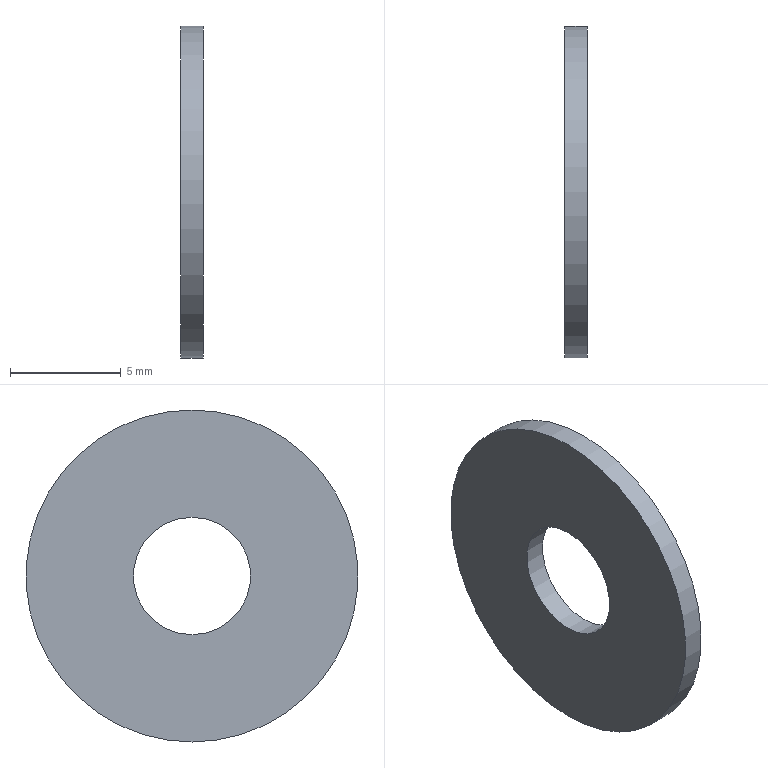Component | NX | GB-T96_1-2002_M5 | 1 solid | 4 faces | box 1 x 15 x 15 mm | volume 155 mm3 | cylinder 2 | plane 2 | commonest cylinder face diameters 15 x1 5.3 x1
STEP:
#1=CARTESIAN_POINT('',(0.,0.,0.));
#2=DIRECTION('',(0.,0.,1.));
#3=DIRECTION('',(1.,0.,0.));
#4=AXIS2_PLACEMENT_3D('',#1,#2,#3);
#5=CARTESIAN_POINT('',(16.,-0.,39.5));
#6=VERTEX_POINT('',#5);
#7=CARTESIAN_POINT('',(16.,-0.,32.));
#8=DIRECTION('',(-1.,0.,0.));
#9=DIRECTION('',(0.,0.,1.));
#10=AXIS2_PLACEMENT_3D('',#7,#8,#9);
#11=CIRCLE('',#10,7.5);
#12=CARTESIAN_POINT('',(16.,-0.,32.));
#13=DIRECTION('',(1.,0.,0.));
#14=DIRECTION('',(0.,0.,-1.));
#15=AXIS2_PLACEMENT_3D('',#12,#13,#14);
#16=CYLINDRICAL_SURFACE('',#15,7.5);
#17=CARTESIAN_POINT('',(9.425,0.));
#18=DIRECTION('',(-1.,0.));
#19=VECTOR('',#18,1.);
#20=LINE('',#17,#19);
#21=(GEOMETRIC_REPRESENTATION_CONTEXT(2)PARAMETRIC_REPRESENTATION_CONTEXT()REPRESENTATION_CONTEXT('',''));
#22=DEFINITIONAL_REPRESENTATION('',(#20),#21);
#23=PCURVE('',#16,#22);
#24=CARTESIAN_POINT('',(16.,-0.,32.));
#25=DIRECTION('',(-1.,0.,0.));
#26=DIRECTION('',(0.,0.,1.));
#27=AXIS2_PLACEMENT_3D('',#24,#25,#26);
#28=PLANE('',#27);
#29=CARTESIAN_POINT('',(0.,0.));
#30=DIRECTION('',(1.,0.));
#31=AXIS2_PLACEMENT_2D('',#29,#30);
#32=CIRCLE('',#31,7.5);
#33=(GEOMETRIC_REPRESENTATION_CONTEXT(2)PARAMETRIC_REPRESENTATION_CONTEXT()REPRESENTATION_CONTEXT('',''));
#34=DEFINITIONAL_REPRESENTATION('',(#32),#33);
#35=PCURVE('',#28,#34);
#36=SURFACE_CURVE('',#11,(#23,#35),.PCURVE_S1.);
#37=EDGE_CURVE('',#6,#6,#36,.T.);
#38=ORIENTED_EDGE('',*,*,#37,.F.);
#39=CARTESIAN_POINT('',(17.,-0.,39.5));
#40=VERTEX_POINT('',#39);
#41=CARTESIAN_POINT('',(16.,-0.,39.5));
#42=CARTESIAN_POINT('',(17.,-0.,39.5));
#43=B_SPLINE_CURVE_WITH_KNOTS('',1,(#41,#42),.UNSPECIFIED.,.F.,.F.,(2,2),(0.,1.),.PIECEWISE_BEZIER_KNOTS.);
#44=CARTESIAN_POINT('',(9.425,0.));
#45=DIRECTION('',(0.,1.));
#46=VECTOR('',#45,1.);
#47=LINE('',#44,#46);
#48=(GEOMETRIC_REPRESENTATION_CONTEXT(2)PARAMETRIC_REPRESENTATION_CONTEXT()REPRESENTATION_CONTEXT('',''));
#49=DEFINITIONAL_REPRESENTATION('',(#47),#48);
#50=PCURVE('',#16,#49);
#51=CARTESIAN_POINT('',(3.142,0.));
#52=DIRECTION('',(0.,1.));
#53=VECTOR('',#52,1.);
#54=LINE('',#51,#53);
#55=(GEOMETRIC_REPRESENTATION_CONTEXT(2)PARAMETRIC_REPRESENTATION_CONTEXT()REPRESENTATION_CONTEXT('',''));
#56=DEFINITIONAL_REPRESENTATION('',(#54),#55);
#57=PCURVE('',#16,#56);
#58=SEAM_CURVE('',#43,(#50,#57),.PCURVE_S1.);
#59=EDGE_CURVE('',#6,#40,#58,.T.);
#60=ORIENTED_EDGE('',*,*,#59,.T.);
#61=CARTESIAN_POINT('',(17.,-0.,32.));
#62=DIRECTION('',(-1.,0.,0.));
#63=DIRECTION('',(0.,0.,1.));
#64=AXIS2_PLACEMENT_3D('',#61,#62,#63);
#65=CIRCLE('',#64,7.5);
#66=CARTESIAN_POINT('',(9.425,1.));
#67=DIRECTION('',(-1.,0.));
#68=VECTOR('',#67,1.);
#69=LINE('',#66,#68);
#70=(GEOMETRIC_REPRESENTATION_CONTEXT(2)PARAMETRIC_REPRESENTATION_CONTEXT()REPRESENTATION_CONTEXT('',''));
#71=DEFINITIONAL_REPRESENTATION('',(#69),#70);
#72=PCURVE('',#16,#71);
#73=CARTESIAN_POINT('',(17.,-0.,32.));
#74=DIRECTION('',(-1.,0.,0.));
#75=DIRECTION('',(0.,0.,1.));
#76=AXIS2_PLACEMENT_3D('',#73,#74,#75);
#77=PLANE('',#76);
#78=CARTESIAN_POINT('',(0.,0.));
#79=DIRECTION('',(1.,0.));
#80=AXIS2_PLACEMENT_2D('',#78,#79);
#81=CIRCLE('',#80,7.5);
#82=(GEOMETRIC_REPRESENTATION_CONTEXT(2)PARAMETRIC_REPRESENTATION_CONTEXT()REPRESENTATION_CONTEXT('',''));
#83=DEFINITIONAL_REPRESENTATION('',(#81),#82);
#84=PCURVE('',#77,#83);
#85=SURFACE_CURVE('',#65,(#72,#84),.PCURVE_S1.);
#86=EDGE_CURVE('',#40,#40,#85,.T.);
#87=ORIENTED_EDGE('',*,*,#86,.T.);
#88=ORIENTED_EDGE('',*,*,#59,.F.);
#89=EDGE_LOOP('',(#38,#60,#87,#88));
#90=FACE_BOUND('',#89,.T.);
#91=ADVANCED_FACE('',(#90),#16,.T.);
#92=CARTESIAN_POINT('',(16.,-0.,34.65));
#93=VERTEX_POINT('',#92);
#94=CARTESIAN_POINT('',(16.,-0.,32.));
#95=DIRECTION('',(-1.,0.,0.));
#96=DIRECTION('',(0.,0.,1.));
#97=AXIS2_PLACEMENT_3D('',#94,#95,#96);
#98=CIRCLE('',#97,2.65);
#99=CARTESIAN_POINT('',(16.,-0.,32.));
#100=DIRECTION('',(1.,0.,0.));
#101=DIRECTION('',(0.,0.,-1.));
#102=AXIS2_PLACEMENT_3D('',#99,#100,#101);
#103=CYLINDRICAL_SURFACE('',#102,2.65);
#104=CARTESIAN_POINT('',(9.425,0.));
#105=DIRECTION('',(-1.,0.));
#106=VECTOR('',#105,1.);
#107=LINE('',#104,#106);
#108=(GEOMETRIC_REPRESENTATION_CONTEXT(2)PARAMETRIC_REPRESENTATION_CONTEXT()REPRESENTATION_CONTEXT('',''));
#109=DEFINITIONAL_REPRESENTATION('',(#107),#108);
#110=PCURVE('',#103,#109);
#111=CARTESIAN_POINT('',(0.,0.));
#112=DIRECTION('',(1.,0.));
#113=AXIS2_PLACEMENT_2D('',#111,#112);
#114=CIRCLE('',#113,2.65);
#115=(GEOMETRIC_REPRESENTATION_CONTEXT(2)PARAMETRIC_REPRESENTATION_CONTEXT()REPRESENTATION_CONTEXT('',''));
#116=DEFINITIONAL_REPRESENTATION('',(#114),#115);
#117=PCURVE('',#28,#116);
#118=SURFACE_CURVE('',#98,(#110,#117),.PCURVE_S1.);
#119=EDGE_CURVE('',#93,#93,#118,.T.);
#120=ORIENTED_EDGE('',*,*,#119,.F.);
#121=CARTESIAN_POINT('',(17.,-0.,34.65));
#122=VERTEX_POINT('',#121);
#123=CARTESIAN_POINT('',(16.,-0.,34.65));
#124=CARTESIAN_POINT('',(17.,-0.,34.65));
#125=B_SPLINE_CURVE_WITH_KNOTS('',1,(#123,#124),.UNSPECIFIED.,.F.,.F.,(2,2),(0.,1.),.PIECEWISE_BEZIER_KNOTS.);
#126=CARTESIAN_POINT('',(9.425,0.));
#127=DIRECTION('',(0.,1.));
#128=VECTOR('',#127,1.);
#129=LINE('',#126,#128);
#130=(GEOMETRIC_REPRESENTATION_CONTEXT(2)PARAMETRIC_REPRESENTATION_CONTEXT()REPRESENTATION_CONTEXT('',''));
#131=DEFINITIONAL_REPRESENTATION('',(#129),#130);
#132=PCURVE('',#103,#131);
#133=CARTESIAN_POINT('',(3.142,0.));
#134=DIRECTION('',(0.,1.));
#135=VECTOR('',#134,1.);
#136=LINE('',#133,#135);
#137=(GEOMETRIC_REPRESENTATION_CONTEXT(2)PARAMETRIC_REPRESENTATION_CONTEXT()REPRESENTATION_CONTEXT('',''));
#138=DEFINITIONAL_REPRESENTATION('',(#136),#137);
#139=PCURVE('',#103,#138);
#140=SEAM_CURVE('',#125,(#132,#139),.PCURVE_S1.);
#141=EDGE_CURVE('',#93,#122,#140,.T.);
#142=ORIENTED_EDGE('',*,*,#141,.T.);
#143=CARTESIAN_POINT('',(17.,-0.,32.));
#144=DIRECTION('',(-1.,0.,0.));
#145=DIRECTION('',(0.,0.,1.));
#146=AXIS2_PLACEMENT_3D('',#143,#144,#145);
#147=CIRCLE('',#146,2.65);
#148=CARTESIAN_POINT('',(9.425,1.));
#149=DIRECTION('',(-1.,0.));
#150=VECTOR('',#149,1.);
#151=LINE('',#148,#150);
#152=(GEOMETRIC_REPRESENTATION_CONTEXT(2)PARAMETRIC_REPRESENTATION_CONTEXT()REPRESENTATION_CONTEXT('',''));
#153=DEFINITIONAL_REPRESENTATION('',(#151),#152);
#154=PCURVE('',#103,#153);
#155=CARTESIAN_POINT('',(0.,0.));
#156=DIRECTION('',(1.,0.));
#157=AXIS2_PLACEMENT_2D('',#155,#156);
#158=CIRCLE('',#157,2.65);
#159=(GEOMETRIC_REPRESENTATION_CONTEXT(2)PARAMETRIC_REPRESENTATION_CONTEXT()REPRESENTATION_CONTEXT('',''));
#160=DEFINITIONAL_REPRESENTATION('',(#158),#159);
#161=PCURVE('',#77,#160);
#162=SURFACE_CURVE('',#147,(#154,#161),.PCURVE_S1.);
#163=EDGE_CURVE('',#122,#122,#162,.T.);
#164=ORIENTED_EDGE('',*,*,#163,.T.);
#165=ORIENTED_EDGE('',*,*,#141,.F.);
#166=EDGE_LOOP('',(#120,#142,#164,#165));
#167=FACE_BOUND('',#166,.F.);
#168=ADVANCED_FACE('',(#167),#103,.F.);
#169=ORIENTED_EDGE('',*,*,#37,.T.);
#170=EDGE_LOOP('',(#169));
#171=FACE_BOUND('',#170,.T.);
#172=ORIENTED_EDGE('',*,*,#119,.F.);
#173=EDGE_LOOP('',(#172));
#174=FACE_BOUND('',#173,.T.);
#175=ADVANCED_FACE('',(#171,#174),#28,.T.);
#176=ORIENTED_EDGE('',*,*,#86,.F.);
#177=EDGE_LOOP('',(#176));
#178=FACE_BOUND('',#177,.T.);
#179=ORIENTED_EDGE('',*,*,#163,.T.);
#180=EDGE_LOOP('',(#179));
#181=FACE_BOUND('',#180,.T.);
#182=ADVANCED_FACE('',(#178,#181),#77,.F.);
#183=CLOSED_SHELL('',(#91,#168,#175,#182));
#184=MANIFOLD_SOLID_BREP('',#183);
#185=(LENGTH_UNIT()NAMED_UNIT(*)SI_UNIT(.MILLI.,.METRE.));
#186=UNCERTAINTY_MEASURE_WITH_UNIT(LENGTH_MEASURE(0.00001),#185,'','');
#187=(NAMED_UNIT(*)PLANE_ANGLE_UNIT()SI_UNIT($,.RADIAN.));
#188=(NAMED_UNIT(*)SI_UNIT($,.STERADIAN.)SOLID_ANGLE_UNIT());
#189=(GEOMETRIC_REPRESENTATION_CONTEXT(3)GLOBAL_UNCERTAINTY_ASSIGNED_CONTEXT((#186))GLOBAL_UNIT_ASSIGNED_CONTEXT((#185,#187,#188))REPRESENTATION_CONTEXT('',''));
#190=ADVANCED_BREP_SHAPE_REPRESENTATION('',(#4,#184),#189);